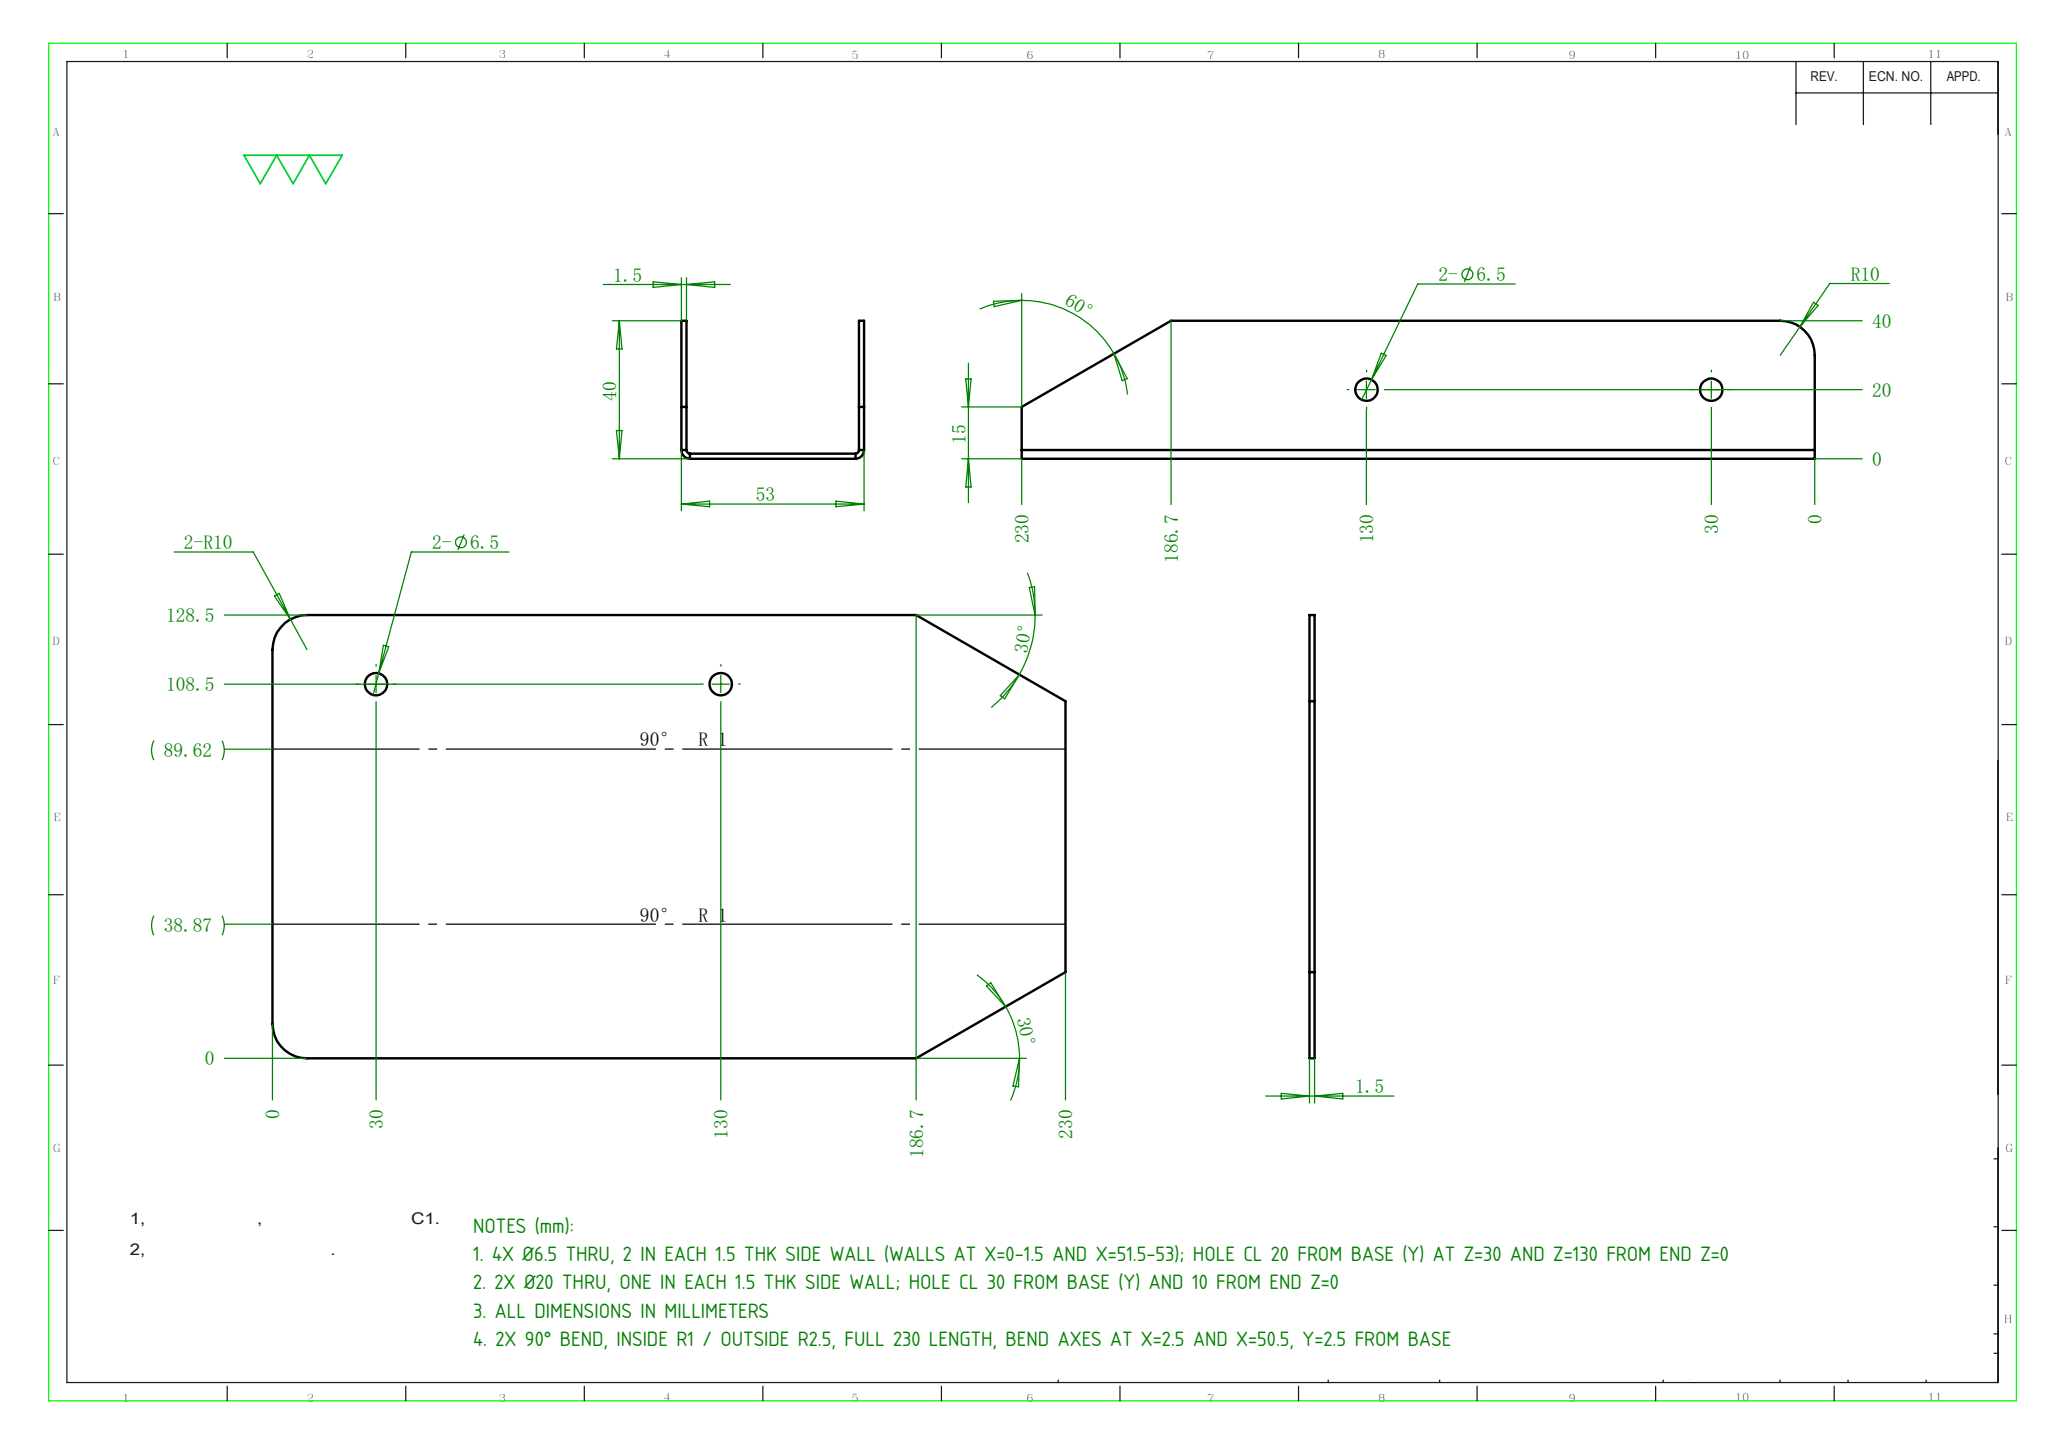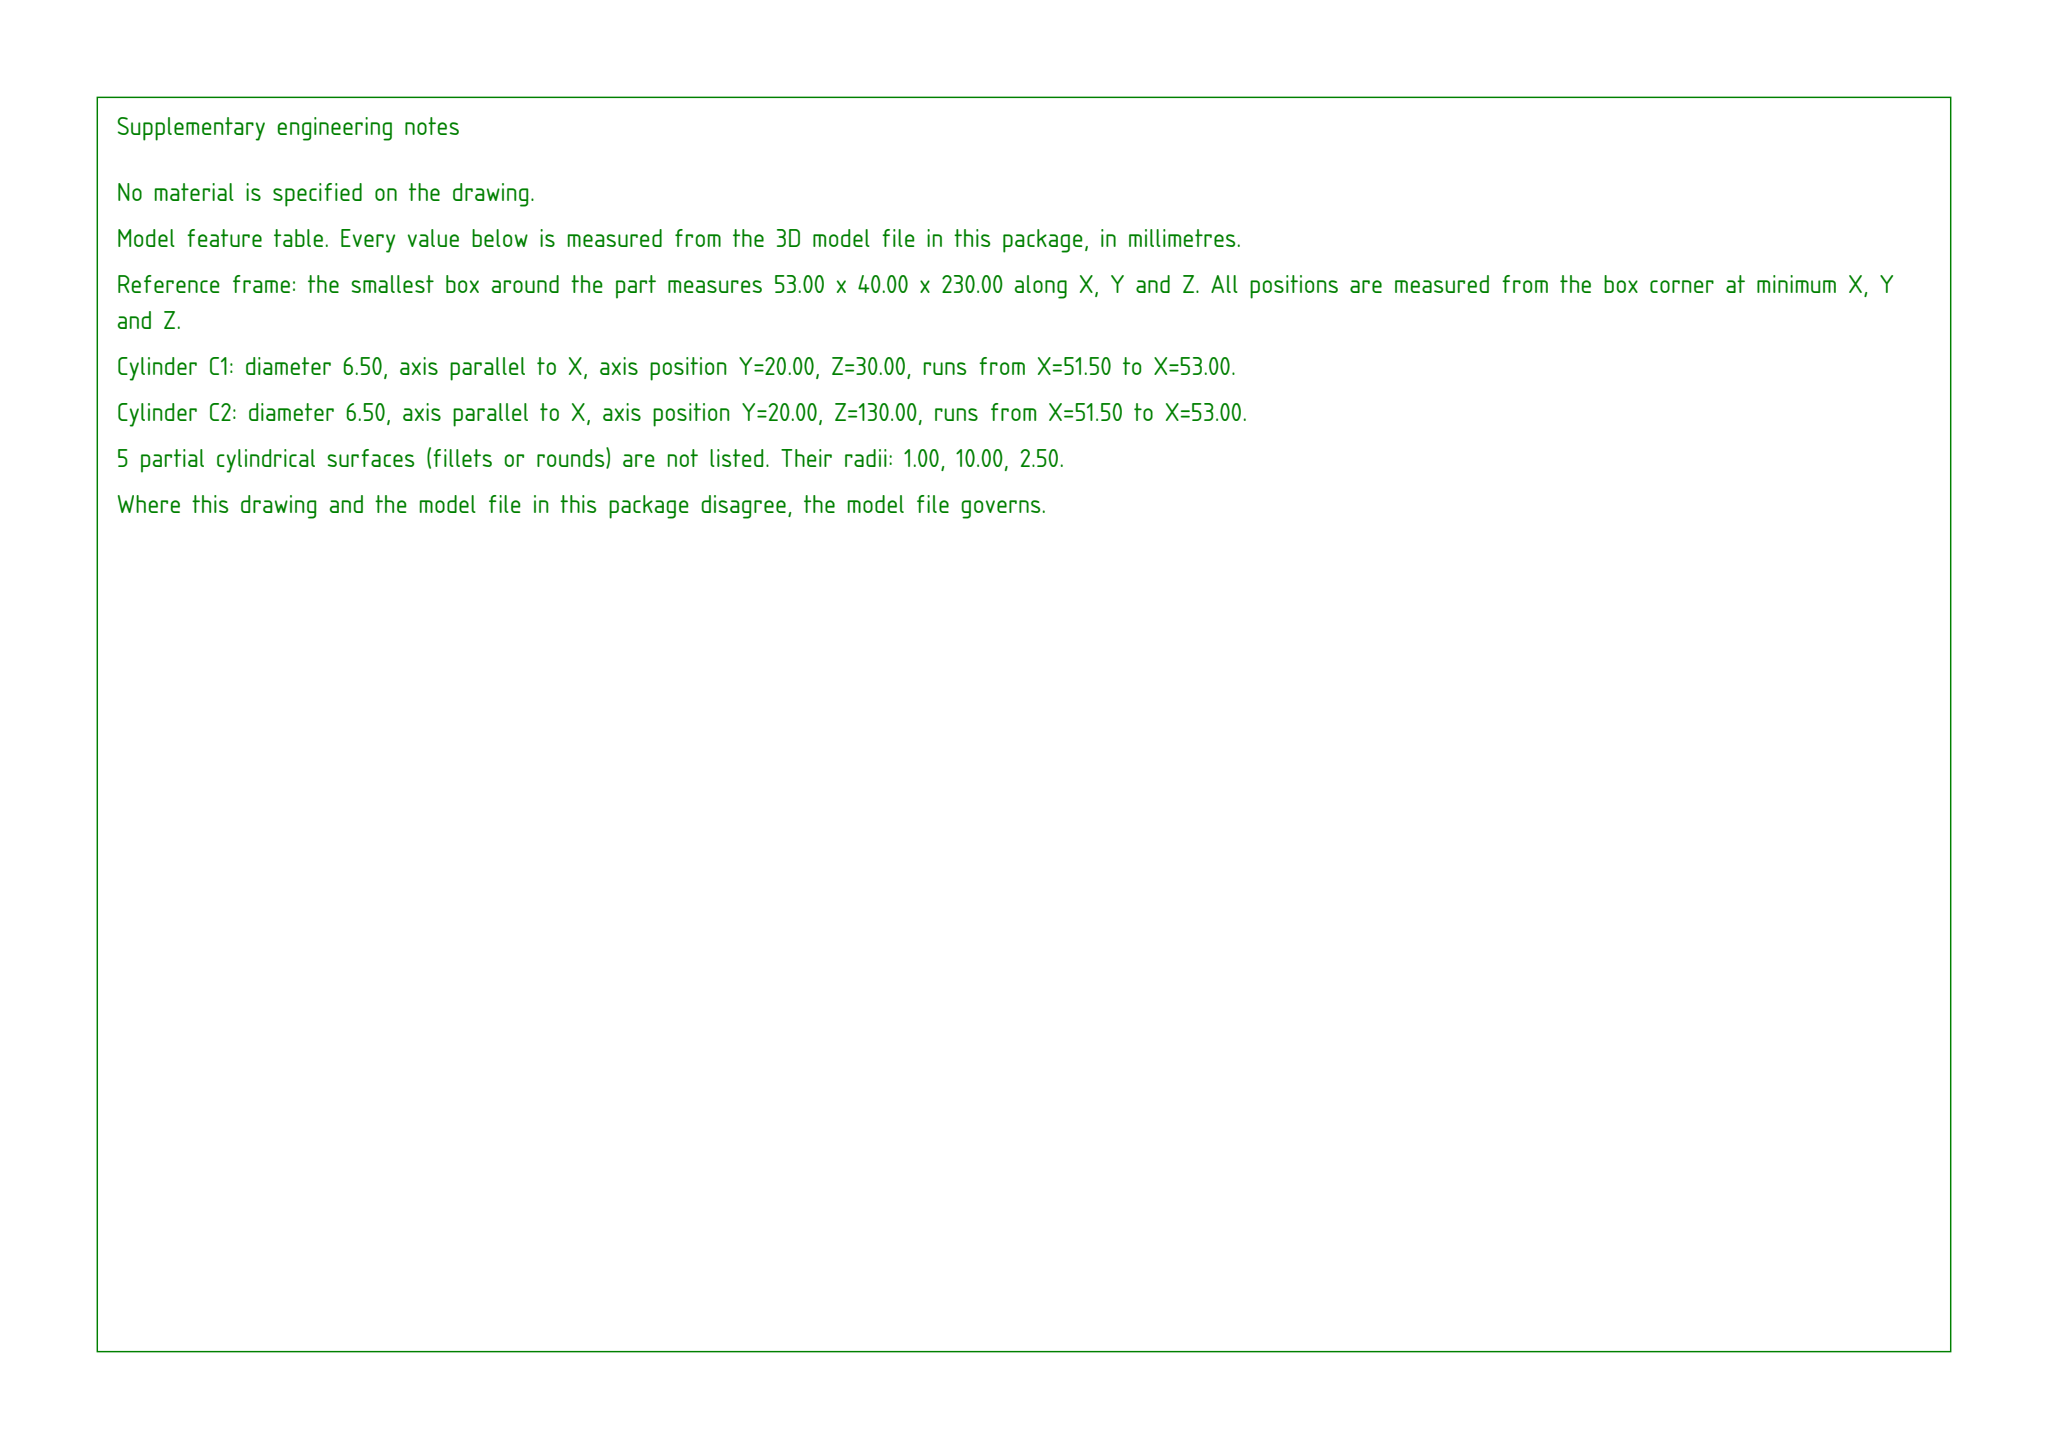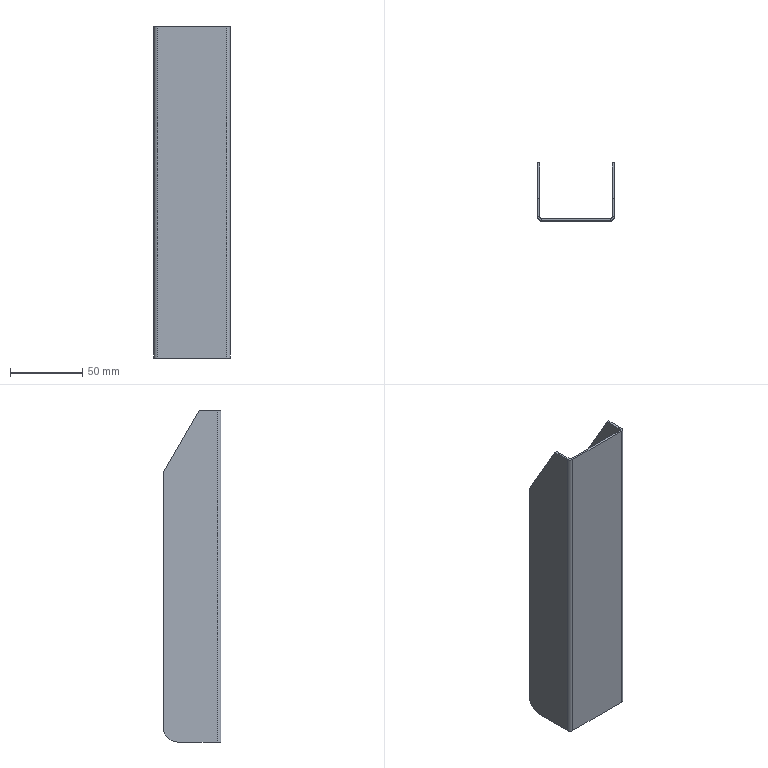Part | SolidWorks | mm | 1 solid | 30 faces | box 53 x 40 x 230 mm | volume 42544 mm3 | plane 20 | cylinder 10 | commonest cylinder face diameters 6.5 x4 2 x2 5 x2 20 x2
Drawing notes:
4X Ø6.5 THRU, 2 IN EACH 1.5 THK SIDE WALL (WALLS AT X=0-1.5 AND X=51.5-53); HOLE CL 20 FROM BASE (Y) AT Z=30 AND Z=130 FROM END Z=0 | from the solid: cylinders dia 6.5, axis x, [null,20,30] and [null,20,130], length 1.5, count 2 each
2X Ø20 THRU, ONE IN EACH 1.5 THK SIDE WALL; HOLE CL 30 FROM BASE (Y) AND 10 FROM END Z=0 | from the solid: cylinders dia 20, axis x, [null,30,10], length 1.5, count 2
ALL DIMENSIONS IN MILLIMETERS | from the solid: STEP model bbox and all feature sizes given in mm (53 x 40 x 230)
2X 90° BEND, INSIDE R1 / OUTSIDE R2.5, FULL 230 LENGTH, BEND AXES AT X=2.5 AND X=50.5, Y=2.5 FROM BASE | from the solid: cylinders dia 2.0 and dia 5.0, axis z, at (x=2.5,y=2.5) and (x=50.5,y=2.5), length 230
STEP:
#1=CARTESIAN_POINT('',(51.5,18.5,-193.25));
#2=VERTEX_POINT('',#1);
#3=CARTESIAN_POINT('',(51.5,18.5,-186.75));
#4=VERTEX_POINT('',#3);
#5=CARTESIAN_POINT('',(51.5,18.5,-190.));
#6=DIRECTION('',(-1.,0.,0.));
#7=DIRECTION('',(0.,0.,1.));
#8=AXIS2_PLACEMENT_3D('',#5,#6,#7);
#9=CIRCLE('',#8,3.25);
#10=EDGE_CURVE('',#2,#4,#9,.T.);
#11=ORIENTED_EDGE('',*,*,#10,.F.);
#12=CARTESIAN_POINT('',(50.,18.5,-193.25));
#13=VERTEX_POINT('',#12);
#14=CARTESIAN_POINT('',(50.,18.5,-193.25));
#15=DIRECTION('',(-1.,0.,0.));
#16=VECTOR('',#15,1000.);
#17=LINE('',#14,#16);
#18=EDGE_CURVE('',#2,#13,#17,.T.);
#19=ORIENTED_EDGE('',*,*,#18,.T.);
#20=CARTESIAN_POINT('',(50.,18.5,-186.75));
#21=VERTEX_POINT('',#20);
#22=CARTESIAN_POINT('',(50.,18.5,-190.));
#23=DIRECTION('',(-1.,0.,0.));
#24=DIRECTION('',(0.,0.,1.));
#25=AXIS2_PLACEMENT_3D('',#22,#23,#24);
#26=CIRCLE('',#25,3.25);
#27=EDGE_CURVE('',#13,#21,#26,.T.);
#28=ORIENTED_EDGE('',*,*,#27,.T.);
#29=CARTESIAN_POINT('',(50.,18.5,-186.75));
#30=DIRECTION('',(-1.,0.,0.));
#31=VECTOR('',#30,1000.);
#32=LINE('',#29,#31);
#33=EDGE_CURVE('',#4,#21,#32,.T.);
#34=ORIENTED_EDGE('',*,*,#33,.F.);
#35=EDGE_LOOP('',(#11,#19,#28,#34));
#36=FACE_OUTER_BOUND('',#35,.T.);
#37=CARTESIAN_POINT('',(50.,18.5,-190.));
#38=DIRECTION('',(-1.,0.,0.));
#39=DIRECTION('',(0.,0.,1.));
#40=AXIS2_PLACEMENT_3D('',#37,#38,#39);
#41=CYLINDRICAL_SURFACE('',#40,3.25);
#42=ADVANCED_FACE('',(#36),#41,.F.);
#43=CARTESIAN_POINT('',(51.5,18.5,-93.25));
#44=VERTEX_POINT('',#43);
#45=CARTESIAN_POINT('',(51.5,18.5,-86.75));
#46=VERTEX_POINT('',#45);
#47=CARTESIAN_POINT('',(51.5,18.5,-90.));
#48=DIRECTION('',(-1.,0.,0.));
#49=DIRECTION('',(0.,0.,1.));
#50=AXIS2_PLACEMENT_3D('',#47,#48,#49);
#51=CIRCLE('',#50,3.25);
#52=EDGE_CURVE('',#44,#46,#51,.T.);
#53=ORIENTED_EDGE('',*,*,#52,.F.);
#54=CARTESIAN_POINT('',(50.,18.5,-93.25));
#55=VERTEX_POINT('',#54);
#56=CARTESIAN_POINT('',(50.,18.5,-93.25));
#57=DIRECTION('',(-1.,0.,0.));
#58=VECTOR('',#57,1000.);
#59=LINE('',#56,#58);
#60=EDGE_CURVE('',#44,#55,#59,.T.);
#61=ORIENTED_EDGE('',*,*,#60,.T.);
#62=CARTESIAN_POINT('',(50.,18.5,-86.75));
#63=VERTEX_POINT('',#62);
#64=CARTESIAN_POINT('',(50.,18.5,-90.));
#65=DIRECTION('',(-1.,0.,0.));
#66=DIRECTION('',(0.,0.,1.));
#67=AXIS2_PLACEMENT_3D('',#64,#65,#66);
#68=CIRCLE('',#67,3.25);
#69=EDGE_CURVE('',#55,#63,#68,.T.);
#70=ORIENTED_EDGE('',*,*,#69,.T.);
#71=CARTESIAN_POINT('',(50.,18.5,-86.75));
#72=DIRECTION('',(-1.,0.,0.));
#73=VECTOR('',#72,1000.);
#74=LINE('',#71,#73);
#75=EDGE_CURVE('',#46,#63,#74,.T.);
#76=ORIENTED_EDGE('',*,*,#75,.F.);
#77=EDGE_LOOP('',(#53,#61,#70,#76));
#78=FACE_OUTER_BOUND('',#77,.T.);
#79=CARTESIAN_POINT('',(50.,18.5,-90.));
#80=DIRECTION('',(-1.,0.,0.));
#81=DIRECTION('',(0.,0.,1.));
#82=AXIS2_PLACEMENT_3D('',#79,#80,#81);
#83=CYLINDRICAL_SURFACE('',#82,3.25);
#84=ADVANCED_FACE('',(#78),#83,.F.);
#85=CARTESIAN_POINT('',(51.5,1.,10.));
#86=VERTEX_POINT('',#85);
#87=CARTESIAN_POINT('',(51.5,13.5,10.));
#88=VERTEX_POINT('',#87);
#89=CARTESIAN_POINT('',(51.5,0.,10.));
#90=DIRECTION('',(0.,1.,0.));
#91=VECTOR('',#90,1000.);
#92=LINE('',#89,#91);
#93=EDGE_CURVE('',#86,#88,#92,.T.);
#94=ORIENTED_EDGE('',*,*,#93,.T.);
#95=CARTESIAN_POINT('',(50.,13.5,10.));
#96=VERTEX_POINT('',#95);
#97=CARTESIAN_POINT('',(50.,13.5,10.));
#98=DIRECTION('',(1.,0.,0.));
#99=VECTOR('',#98,1000.);
#100=LINE('',#97,#99);
#101=EDGE_CURVE('',#96,#88,#100,.T.);
#102=ORIENTED_EDGE('',*,*,#101,.F.);
#103=CARTESIAN_POINT('',(50.,1.,10.));
#104=VERTEX_POINT('',#103);
#105=CARTESIAN_POINT('',(50.,0.,10.));
#106=DIRECTION('',(0.,1.,0.));
#107=VECTOR('',#106,1000.);
#108=LINE('',#105,#107);
#109=EDGE_CURVE('',#104,#96,#108,.T.);
#110=ORIENTED_EDGE('',*,*,#109,.F.);
#111=CARTESIAN_POINT('',(50.,1.,10.));
#112=DIRECTION('',(1.,0.,0.));
#113=VECTOR('',#112,1000.);
#114=LINE('',#111,#113);
#115=EDGE_CURVE('',#104,#86,#114,.T.);
#116=ORIENTED_EDGE('',*,*,#115,.T.);
#117=EDGE_LOOP('',(#94,#102,#110,#116));
#118=FACE_OUTER_BOUND('',#117,.T.);
#119=CARTESIAN_POINT('',(49.,-1.5,10.));
#120=DIRECTION('',(0.,0.,1.));
#121=DIRECTION('',(1.,0.,0.));
#122=AXIS2_PLACEMENT_3D('',#119,#120,#121);
#123=PLANE('',#122);
#124=ADVANCED_FACE('',(#118),#123,.T.);
#125=CARTESIAN_POINT('',(51.5,18.5,-90.));
#126=DIRECTION('',(-1.,0.,0.));
#127=DIRECTION('',(0.,0.,1.));
#128=AXIS2_PLACEMENT_3D('',#125,#126,#127);
#129=CIRCLE('',#128,3.25);
#130=EDGE_CURVE('',#46,#44,#129,.T.);
#131=ORIENTED_EDGE('',*,*,#130,.T.);
#132=ORIENTED_EDGE('',*,*,#52,.T.);
#133=EDGE_LOOP('',(#131,#132));
#134=FACE_BOUND('',#133,.T.);
#135=CARTESIAN_POINT('',(51.5,18.5,-190.));
#136=DIRECTION('',(-1.,0.,0.));
#137=DIRECTION('',(0.,0.,1.));
#138=AXIS2_PLACEMENT_3D('',#135,#136,#137);
#139=CIRCLE('',#138,3.25);
#140=EDGE_CURVE('',#4,#2,#139,.T.);
#141=ORIENTED_EDGE('',*,*,#140,.T.);
#142=ORIENTED_EDGE('',*,*,#10,.T.);
#143=EDGE_LOOP('',(#141,#142));
#144=FACE_BOUND('',#143,.T.);
#145=CARTESIAN_POINT('',(51.5,38.5,-33.301));
#146=VERTEX_POINT('',#145);
#147=CARTESIAN_POINT('',(51.5,10.125,15.846));
#148=DIRECTION('',(0.,-0.5,0.866));
#149=VECTOR('',#148,1000.);
#150=LINE('',#147,#149);
#151=EDGE_CURVE('',#146,#88,#150,.T.);
#152=ORIENTED_EDGE('',*,*,#151,.T.);
#153=ORIENTED_EDGE('',*,*,#93,.F.);
#154=CARTESIAN_POINT('',(51.5,1.,-220.));
#155=VERTEX_POINT('',#154);
#156=CARTESIAN_POINT('',(51.5,1.,10.));
#157=DIRECTION('',(0.,0.,-1.));
#158=VECTOR('',#157,1000.);
#159=LINE('',#156,#158);
#160=EDGE_CURVE('',#86,#155,#159,.T.);
#161=ORIENTED_EDGE('',*,*,#160,.T.);
#162=CARTESIAN_POINT('',(51.5,28.5,-220.));
#163=VERTEX_POINT('',#162);
#164=CARTESIAN_POINT('',(51.5,0.,-220.));
#165=DIRECTION('',(0.,1.,0.));
#166=VECTOR('',#165,1000.);
#167=LINE('',#164,#166);
#168=EDGE_CURVE('',#155,#163,#167,.T.);
#169=ORIENTED_EDGE('',*,*,#168,.T.);
#170=CARTESIAN_POINT('',(51.5,38.5,-210.));
#171=VERTEX_POINT('',#170);
#172=CARTESIAN_POINT('',(51.5,28.5,-210.));
#173=DIRECTION('',(1.,0.,0.));
#174=DIRECTION('',(0.,0.,1.));
#175=AXIS2_PLACEMENT_3D('',#172,#173,#174);
#176=CIRCLE('',#175,10.);
#177=EDGE_CURVE('',#163,#171,#176,.T.);
#178=ORIENTED_EDGE('',*,*,#177,.T.);
#179=CARTESIAN_POINT('',(51.5,38.5,10.));
#180=DIRECTION('',(0.,0.,-1.));
#181=VECTOR('',#180,1000.);
#182=LINE('',#179,#181);
#183=EDGE_CURVE('',#146,#171,#182,.T.);
#184=ORIENTED_EDGE('',*,*,#183,.F.);
#185=EDGE_LOOP('',(#152,#153,#161,#169,#178,#184));
#186=FACE_OUTER_BOUND('',#185,.T.);
#187=CARTESIAN_POINT('',(51.5,0.,10.));
#188=DIRECTION('',(-1.,0.,0.));
#189=DIRECTION('',(0.,0.,1.));
#190=AXIS2_PLACEMENT_3D('',#187,#188,#189);
#191=PLANE('',#190);
#192=ADVANCED_FACE('',(#134,#144,#186),#191,.F.);
#193=CARTESIAN_POINT('',(50.,38.5,-33.301));
#194=VERTEX_POINT('',#193);
#195=CARTESIAN_POINT('',(50.,38.5,-210.));
#196=VERTEX_POINT('',#195);
#197=CARTESIAN_POINT('',(50.,38.5,10.));
#198=DIRECTION('',(0.,0.,-1.));
#199=VECTOR('',#198,1000.);
#200=LINE('',#197,#199);
#201=EDGE_CURVE('',#194,#196,#200,.T.);
#202=ORIENTED_EDGE('',*,*,#201,.F.);
#203=CARTESIAN_POINT('',(50.,38.5,-33.301));
#204=DIRECTION('',(1.,0.,0.));
#205=VECTOR('',#204,1000.);
#206=LINE('',#203,#205);
#207=EDGE_CURVE('',#194,#146,#206,.T.);
#208=ORIENTED_EDGE('',*,*,#207,.T.);
#209=ORIENTED_EDGE('',*,*,#183,.T.);
#210=CARTESIAN_POINT('',(50.,38.5,-210.));
#211=DIRECTION('',(-1.,0.,0.));
#212=VECTOR('',#211,1000.);
#213=LINE('',#210,#212);
#214=EDGE_CURVE('',#171,#196,#213,.T.);
#215=ORIENTED_EDGE('',*,*,#214,.T.);
#216=EDGE_LOOP('',(#202,#208,#209,#215));
#217=FACE_OUTER_BOUND('',#216,.T.);
#218=CARTESIAN_POINT('',(50.,38.5,10.));
#219=DIRECTION('',(0.,1.,0.));
#220=DIRECTION('',(0.,0.,1.));
#221=AXIS2_PLACEMENT_3D('',#218,#219,#220);
#222=PLANE('',#221);
#223=ADVANCED_FACE('',(#217),#222,.T.);
#224=CARTESIAN_POINT('',(50.,18.5,-90.));
#225=DIRECTION('',(-1.,0.,0.));
#226=DIRECTION('',(0.,0.,1.));
#227=AXIS2_PLACEMENT_3D('',#224,#225,#226);
#228=CIRCLE('',#227,3.25);
#229=EDGE_CURVE('',#63,#55,#228,.T.);
#230=ORIENTED_EDGE('',*,*,#229,.F.);
#231=ORIENTED_EDGE('',*,*,#69,.F.);
#232=EDGE_LOOP('',(#230,#231));
#233=FACE_BOUND('',#232,.T.);
#234=CARTESIAN_POINT('',(50.,18.5,-190.));
#235=DIRECTION('',(-1.,0.,0.));
#236=DIRECTION('',(0.,0.,1.));
#237=AXIS2_PLACEMENT_3D('',#234,#235,#236);
#238=CIRCLE('',#237,3.25);
#239=EDGE_CURVE('',#21,#13,#238,.T.);
#240=ORIENTED_EDGE('',*,*,#239,.F.);
#241=ORIENTED_EDGE('',*,*,#27,.F.);
#242=EDGE_LOOP('',(#240,#241));
#243=FACE_BOUND('',#242,.T.);
#244=ORIENTED_EDGE('',*,*,#109,.T.);
#245=CARTESIAN_POINT('',(50.,10.125,15.846));
#246=DIRECTION('',(0.,-0.5,0.866));
#247=VECTOR('',#246,1000.);
#248=LINE('',#245,#247);
#249=EDGE_CURVE('',#194,#96,#248,.T.);
#250=ORIENTED_EDGE('',*,*,#249,.F.);
#251=ORIENTED_EDGE('',*,*,#201,.T.);
#252=CARTESIAN_POINT('',(50.,28.5,-220.));
#253=VERTEX_POINT('',#252);
#254=CARTESIAN_POINT('',(50.,28.5,-210.));
#255=DIRECTION('',(-1.,0.,0.));
#256=DIRECTION('',(0.,0.,1.));
#257=AXIS2_PLACEMENT_3D('',#254,#255,#256);
#258=CIRCLE('',#257,10.);
#259=EDGE_CURVE('',#196,#253,#258,.T.);
#260=ORIENTED_EDGE('',*,*,#259,.T.);
#261=CARTESIAN_POINT('',(50.,1.,-220.));
#262=VERTEX_POINT('',#261);
#263=CARTESIAN_POINT('',(50.,0.,-220.));
#264=DIRECTION('',(0.,1.,0.));
#265=VECTOR('',#264,1000.);
#266=LINE('',#263,#265);
#267=EDGE_CURVE('',#262,#253,#266,.T.);
#268=ORIENTED_EDGE('',*,*,#267,.F.);
#269=CARTESIAN_POINT('',(50.,1.,10.));
#270=DIRECTION('',(0.,0.,-1.));
#271=VECTOR('',#270,1000.);
#272=LINE('',#269,#271);
#273=EDGE_CURVE('',#104,#262,#272,.T.);
#274=ORIENTED_EDGE('',*,*,#273,.F.);
#275=EDGE_LOOP('',(#244,#250,#251,#260,#268,#274));
#276=FACE_OUTER_BOUND('',#275,.T.);
#277=CARTESIAN_POINT('',(50.,0.,10.));
#278=DIRECTION('',(-1.,0.,0.));
#279=DIRECTION('',(0.,0.,1.));
#280=AXIS2_PLACEMENT_3D('',#277,#278,#279);
#281=PLANE('',#280);
#282=ADVANCED_FACE('',(#233,#243,#276),#281,.T.);
#283=CARTESIAN_POINT('',(0.,38.5,-33.301));
#284=VERTEX_POINT('',#283);
#285=CARTESIAN_POINT('',(0.,38.5,-210.));
#286=VERTEX_POINT('',#285);
#287=CARTESIAN_POINT('',(0.,38.5,10.));
#288=DIRECTION('',(0.,0.,-1.));
#289=VECTOR('',#288,1000.);
#290=LINE('',#287,#289);
#291=EDGE_CURVE('',#284,#286,#290,.T.);
#292=ORIENTED_EDGE('',*,*,#291,.F.);
#293=CARTESIAN_POINT('',(0.,13.5,10.));
#294=VERTEX_POINT('',#293);
#295=CARTESIAN_POINT('',(0.,10.125,15.846));
#296=DIRECTION('',(0.,0.5,-0.866));
#297=VECTOR('',#296,1000.);
#298=LINE('',#295,#297);
#299=EDGE_CURVE('',#294,#284,#298,.T.);
#300=ORIENTED_EDGE('',*,*,#299,.F.);
#301=CARTESIAN_POINT('',(0.,1.,10.));
#302=VERTEX_POINT('',#301);
#303=CARTESIAN_POINT('',(0.,0.,10.));
#304=DIRECTION('',(0.,-1.,0.));
#305=VECTOR('',#304,1000.);
#306=LINE('',#303,#305);
#307=EDGE_CURVE('',#294,#302,#306,.T.);
#308=ORIENTED_EDGE('',*,*,#307,.T.);
#309=CARTESIAN_POINT('',(0.,1.,-220.));
#310=VERTEX_POINT('',#309);
#311=CARTESIAN_POINT('',(0.,1.,10.));
#312=DIRECTION('',(0.,0.,-1.));
#313=VECTOR('',#312,1000.);
#314=LINE('',#311,#313);
#315=EDGE_CURVE('',#302,#310,#314,.T.);
#316=ORIENTED_EDGE('',*,*,#315,.T.);
#317=CARTESIAN_POINT('',(0.,28.5,-220.));
#318=VERTEX_POINT('',#317);
#319=CARTESIAN_POINT('',(0.,0.,-220.));
#320=DIRECTION('',(0.,-1.,0.));
#321=VECTOR('',#320,1000.);
#322=LINE('',#319,#321);
#323=EDGE_CURVE('',#318,#310,#322,.T.);
#324=ORIENTED_EDGE('',*,*,#323,.F.);
#325=CARTESIAN_POINT('',(0.,28.5,-210.));
#326=DIRECTION('',(1.,0.,0.));
#327=DIRECTION('',(0.,0.,-1.));
#328=AXIS2_PLACEMENT_3D('',#325,#326,#327);
#329=CIRCLE('',#328,10.);
#330=EDGE_CURVE('',#318,#286,#329,.T.);
#331=ORIENTED_EDGE('',*,*,#330,.T.);
#332=EDGE_LOOP('',(#292,#300,#308,#316,#324,#331));
#333=FACE_OUTER_BOUND('',#332,.T.);
#334=CARTESIAN_POINT('',(0.,0.,10.));
#335=DIRECTION('',(1.,0.,0.));
#336=DIRECTION('',(0.,0.,-1.));
#337=AXIS2_PLACEMENT_3D('',#334,#335,#336);
#338=PLANE('',#337);
#339=ADVANCED_FACE('',(#333),#338,.T.);
#340=CARTESIAN_POINT('',(-1.5,38.5,-33.301));
#341=VERTEX_POINT('',#340);
#342=CARTESIAN_POINT('',(-1.5,38.5,-210.));
#343=VERTEX_POINT('',#342);
#344=CARTESIAN_POINT('',(-1.5,38.5,10.));
#345=DIRECTION('',(0.,0.,-1.));
#346=VECTOR('',#345,1000.);
#347=LINE('',#344,#346);
#348=EDGE_CURVE('',#341,#343,#347,.T.);
#349=ORIENTED_EDGE('',*,*,#348,.F.);
#350=CARTESIAN_POINT('',(0.,38.5,-33.301));
#351=DIRECTION('',(-1.,0.,0.));
#352=VECTOR('',#351,1000.);
#353=LINE('',#350,#352);
#354=EDGE_CURVE('',#284,#341,#353,.T.);
#355=ORIENTED_EDGE('',*,*,#354,.F.);
#356=ORIENTED_EDGE('',*,*,#291,.T.);
#357=CARTESIAN_POINT('',(-1.5,38.5,-210.));
#358=DIRECTION('',(-1.,0.,0.));
#359=VECTOR('',#358,1000.);
#360=LINE('',#357,#359);
#361=EDGE_CURVE('',#286,#343,#360,.T.);
#362=ORIENTED_EDGE('',*,*,#361,.T.);
#363=EDGE_LOOP('',(#349,#355,#356,#362));
#364=FACE_OUTER_BOUND('',#363,.T.);
#365=CARTESIAN_POINT('',(-1.5,38.5,10.));
#366=DIRECTION('',(0.,1.,0.));
#367=DIRECTION('',(0.,0.,1.));
#368=AXIS2_PLACEMENT_3D('',#365,#366,#367);
#369=PLANE('',#368);
#370=ADVANCED_FACE('',(#364),#369,.T.);
#371=CARTESIAN_POINT('',(-1.5,13.5,10.));
#372=VERTEX_POINT('',#371);
#373=CARTESIAN_POINT('',(-1.5,10.125,15.846));
#374=DIRECTION('',(0.,0.5,-0.866));
#375=VECTOR('',#374,1000.);
#376=LINE('',#373,#375);
#377=EDGE_CURVE('',#372,#341,#376,.T.);
#378=ORIENTED_EDGE('',*,*,#377,.T.);
#379=ORIENTED_EDGE('',*,*,#348,.T.);
#380=CARTESIAN_POINT('',(-1.5,28.5,-220.));
#381=VERTEX_POINT('',#380);
#382=CARTESIAN_POINT('',(-1.5,28.5,-210.));
#383=DIRECTION('',(-1.,0.,0.));
#384=DIRECTION('',(0.,0.,-1.));
#385=AXIS2_PLACEMENT_3D('',#382,#383,#384);
#386=CIRCLE('',#385,10.);
#387=EDGE_CURVE('',#343,#381,#386,.T.);
#388=ORIENTED_EDGE('',*,*,#387,.T.);
#389=CARTESIAN_POINT('',(-1.5,1.,-220.));
#390=VERTEX_POINT('',#389);
#391=CARTESIAN_POINT('',(-1.5,0.,-220.));
#392=DIRECTION('',(0.,-1.,0.));
#393=VECTOR('',#392,1000.);
#394=LINE('',#391,#393);
#395=EDGE_CURVE('',#381,#390,#394,.T.);
#396=ORIENTED_EDGE('',*,*,#395,.T.);
#397=CARTESIAN_POINT('',(-1.5,1.,10.));
#398=VERTEX_POINT('',#397);
#399=CARTESIAN_POINT('',(-1.5,1.,10.));
#400=DIRECTION('',(0.,0.,-1.));
#401=VECTOR('',#400,1000.);
#402=LINE('',#399,#401);
#403=EDGE_CURVE('',#398,#390,#402,.T.);
#404=ORIENTED_EDGE('',*,*,#403,.F.);
#405=CARTESIAN_POINT('',(-1.5,0.,10.));
#406=DIRECTION('',(0.,-1.,0.));
#407=VECTOR('',#406,1000.);
#408=LINE('',#405,#407);
#409=EDGE_CURVE('',#372,#398,#408,.T.);
#410=ORIENTED_EDGE('',*,*,#409,.F.);
#411=EDGE_LOOP('',(#378,#379,#388,#396,#404,#410));
#412=FACE_OUTER_BOUND('',#411,.T.);
#413=CARTESIAN_POINT('',(-1.5,0.,10.));
#414=DIRECTION('',(1.,0.,0.));
#415=DIRECTION('',(0.,0.,-1.));
#416=AXIS2_PLACEMENT_3D('',#413,#414,#415);
#417=PLANE('',#416);
#418=ADVANCED_FACE('',(#412),#417,.F.);
#419=CARTESIAN_POINT('',(0.,13.5,10.));
#420=DIRECTION('',(-1.,0.,0.));
#421=VECTOR('',#420,1000.);
#422=LINE('',#419,#421);
#423=EDGE_CURVE('',#294,#372,#422,.T.);
#424=ORIENTED_EDGE('',*,*,#423,.T.);
#425=ORIENTED_EDGE('',*,*,#409,.T.);
#426=CARTESIAN_POINT('',(-1.5,1.,10.));
#427=DIRECTION('',(1.,-0.,0.));
#428=VECTOR('',#427,1000.);
#429=LINE('',#426,#428);
#430=EDGE_CURVE('',#398,#302,#429,.T.);
#431=ORIENTED_EDGE('',*,*,#430,.T.);
#432=ORIENTED_EDGE('',*,*,#307,.F.);
#433=EDGE_LOOP('',(#424,#425,#431,#432));
#434=FACE_OUTER_BOUND('',#433,.T.);
#435=CARTESIAN_POINT('',(49.,1.,10.));
#436=DIRECTION('',(0.,0.,-1.));
#437=DIRECTION('',(-1.,0.,0.));
#438=AXIS2_PLACEMENT_3D('',#435,#436,#437);
#439=PLANE('',#438);
#440=ADVANCED_FACE('',(#434),#439,.F.);
#441=CARTESIAN_POINT('',(1.,0.,10.));
#442=VERTEX_POINT('',#441);
#443=CARTESIAN_POINT('',(1.,-1.5,10.));
#444=VERTEX_POINT('',#443);
#445=CARTESIAN_POINT('',(1.,0.,10.));
#446=DIRECTION('',(0.,-1.,0.));
#447=VECTOR('',#446,1000.);
#448=LINE('',#445,#447);
#449=EDGE_CURVE('',#442,#444,#448,.T.);
#450=ORIENTED_EDGE('',*,*,#449,.F.);
#451=CARTESIAN_POINT('',(1.,1.,10.));
#452=DIRECTION('',(0.,0.,1.));
#453=DIRECTION('',(-1.,0.,0.));
#454=AXIS2_PLACEMENT_3D('',#451,#452,#453);
#455=CIRCLE('',#454,1.);
#456=EDGE_CURVE('',#302,#442,#455,.T.);
#457=ORIENTED_EDGE('',*,*,#456,.F.);
#458=ORIENTED_EDGE('',*,*,#430,.F.);
#459=CARTESIAN_POINT('',(1.,1.,10.));
#460=DIRECTION('',(0.,0.,1.));
#461=DIRECTION('',(1.,0.,0.));
#462=AXIS2_PLACEMENT_3D('',#459,#460,#461);
#463=CIRCLE('',#462,2.5);
#464=EDGE_CURVE('',#398,#444,#463,.T.);
#465=ORIENTED_EDGE('',*,*,#464,.T.);
#466=EDGE_LOOP('',(#450,#457,#458,#465));
#467=FACE_OUTER_BOUND('',#466,.T.);
#468=CARTESIAN_POINT('',(1.,0.,10.));
#469=DIRECTION('',(0.,0.,1.));
#470=DIRECTION('',(1.,0.,0.));
#471=AXIS2_PLACEMENT_3D('',#468,#469,#470);
#472=PLANE('',#471);
#473=ADVANCED_FACE('',(#467),#472,.T.);
#474=CARTESIAN_POINT('',(49.,0.,10.));
#475=VERTEX_POINT('',#474);
#476=CARTESIAN_POINT('',(0.,0.,10.));
#477=DIRECTION('',(1.,0.,0.));
#478=VECTOR('',#477,1000.);
#479=LINE('',#476,#478);
#480=EDGE_CURVE('',#442,#475,#479,.T.);
#481=ORIENTED_EDGE('',*,*,#480,.F.);
#482=ORIENTED_EDGE('',*,*,#449,.T.);
#483=CARTESIAN_POINT('',(49.,-1.5,10.));
#484=VERTEX_POINT('',#483);
#485=CARTESIAN_POINT('',(0.,-1.5,10.));
#486=DIRECTION('',(1.,0.,0.));
#487=VECTOR('',#486,1000.);
#488=LINE('',#485,#487);
#489=EDGE_CURVE('',#444,#484,#488,.T.);
#490=ORIENTED_EDGE('',*,*,#489,.T.);
#491=CARTESIAN_POINT('',(49.,-1.5,10.));
#492=DIRECTION('',(0.,1.,0.));
#493=VECTOR('',#492,1000.);
#494=LINE('',#491,#493);
#495=EDGE_CURVE('',#484,#475,#494,.T.);
#496=ORIENTED_EDGE('',*,*,#495,.T.);
#497=EDGE_LOOP('',(#481,#482,#490,#496));
#498=FACE_OUTER_BOUND('',#497,.T.);
#499=CARTESIAN_POINT('',(-1.5,1.,10.));
#500=DIRECTION('',(0.,0.,1.));
#501=DIRECTION('',(1.,0.,0.));
#502=AXIS2_PLACEMENT_3D('',#499,#500,#501);
#503=PLANE('',#502);
#504=ADVANCED_FACE('',(#498),#503,.T.);
#505=CARTESIAN_POINT('',(0.,1.,-220.));
#506=DIRECTION('',(-1.,0.,0.));
#507=VECTOR('',#506,1000.);
#508=LINE('',#505,#507);
#509=EDGE_CURVE('',#310,#390,#508,.T.);
#510=ORIENTED_EDGE('',*,*,#509,.F.);
#511=CARTESIAN_POINT('',(1.,0.,-220.));
#512=VERTEX_POINT('',#511);
#513=CARTESIAN_POINT('',(1.,1.,-220.));
#514=DIRECTION('',(0.,0.,1.));
#515=DIRECTION('',(-1.,0.,0.));
#516=AXIS2_PLACEMENT_3D('',#513,#514,#515);
#517=CIRCLE('',#516,1.);
#518=EDGE_CURVE('',#310,#512,#517,.T.);
#519=ORIENTED_EDGE('',*,*,#518,.T.);
#520=CARTESIAN_POINT('',(1.,-1.5,-220.));
#521=VERTEX_POINT('',#520);
#522=CARTESIAN_POINT('',(1.,-1.5,-220.));
#523=DIRECTION('',(0.,1.,0.));
#524=VECTOR('',#523,1000.);
#525=LINE('',#522,#524);
#526=EDGE_CURVE('',#521,#512,#525,.T.);
#527=ORIENTED_EDGE('',*,*,#526,.F.);
#528=CARTESIAN_POINT('',(1.,1.,-220.));
#529=DIRECTION('',(0.,0.,1.));
#530=DIRECTION('',(1.,0.,0.));
#531=AXIS2_PLACEMENT_3D('',#528,#529,#530);
#532=CIRCLE('',#531,2.5);
#533=EDGE_CURVE('',#390,#521,#532,.T.);
#534=ORIENTED_EDGE('',*,*,#533,.F.);
#535=EDGE_LOOP('',(#510,#519,#527,#534));
#536=FACE_OUTER_BOUND('',#535,.T.);
#537=CARTESIAN_POINT('',(0.,1.,-220.));
#538=DIRECTION('',(0.,0.,-1.));
#539=DIRECTION('',(-1.,0.,0.));
#540=AXIS2_PLACEMENT_3D('',#537,#538,#539);
#541=PLANE('',#540);
#542=ADVANCED_FACE('',(#536),#541,.T.);
#543=ORIENTED_EDGE('',*,*,#395,.F.);
#544=CARTESIAN_POINT('',(1.,28.5,-220.));
#545=DIRECTION('',(1.,0.,0.));
#546=VECTOR('',#545,1000.);
#547=LINE('',#544,#546);
#548=EDGE_CURVE('',#381,#318,#547,.T.);
#549=ORIENTED_EDGE('',*,*,#548,.T.);
#550=ORIENTED_EDGE('',*,*,#323,.T.);
#551=ORIENTED_EDGE('',*,*,#509,.T.);
#552=EDGE_LOOP('',(#543,#549,#550,#551));
#553=FACE_OUTER_BOUND('',#552,.T.);
#554=CARTESIAN_POINT('',(1.,-1.5,-220.));
#555=DIRECTION('',(0.,0.,-1.));
#556=DIRECTION('',(-1.,0.,0.));
#557=AXIS2_PLACEMENT_3D('',#554,#555,#556);
#558=PLANE('',#557);
#559=ADVANCED_FACE('',(#553),#558,.T.);
#560=ORIENTED_EDGE('',*,*,#115,.F.);
#561=CARTESIAN_POINT('',(49.,1.,10.));
#562=DIRECTION('',(0.,0.,1.));
#563=DIRECTION('',(-1.,0.,0.));
#564=AXIS2_PLACEMENT_3D('',#561,#562,#563);
#565=CIRCLE('',#564,1.);
#566=EDGE_CURVE('',#475,#104,#565,.T.);
#567=ORIENTED_EDGE('',*,*,#566,.F.);
#568=ORIENTED_EDGE('',*,*,#495,.F.);
#569=CARTESIAN_POINT('',(49.,1.,10.));
#570=DIRECTION('',(0.,0.,1.));
#571=DIRECTION('',(1.,0.,0.));
#572=AXIS2_PLACEMENT_3D('',#569,#570,#571);
#573=CIRCLE('',#572,2.5);
#574=EDGE_CURVE('',#484,#86,#573,.T.);
#575=ORIENTED_EDGE('',*,*,#574,.T.);
#576=EDGE_LOOP('',(#560,#567,#568,#575));
#577=FACE_OUTER_BOUND('',#576,.T.);
#578=CARTESIAN_POINT('',(50.,1.,10.));
#579=DIRECTION('',(0.,0.,1.));
#580=DIRECTION('',(1.,0.,0.));
#581=AXIS2_PLACEMENT_3D('',#578,#579,#580);
#582=PLANE('',#581);
#583=ADVANCED_FACE('',(#577),#582,.T.);
#584=CARTESIAN_POINT('',(49.,0.,-220.));
#585=VERTEX_POINT('',#584);
#586=CARTESIAN_POINT('',(49.,-1.5,-220.));
#587=VERTEX_POINT('',#586);
#588=CARTESIAN_POINT('',(49.,0.,-220.));
#589=DIRECTION('',(0.,-1.,0.));
#590=VECTOR('',#589,1000.);
#591=LINE('',#588,#590);
#592=EDGE_CURVE('',#585,#587,#591,.T.);
#593=ORIENTED_EDGE('',*,*,#592,.F.);
#594=CARTESIAN_POINT('',(49.,1.,-220.));
#595=DIRECTION('',(0.,0.,1.));
#596=DIRECTION('',(-1.,0.,0.));
#597=AXIS2_PLACEMENT_3D('',#594,#595,#596);
#598=CIRCLE('',#597,1.);
#599=EDGE_CURVE('',#585,#262,#598,.T.);
#600=ORIENTED_EDGE('',*,*,#599,.T.);
#601=CARTESIAN_POINT('',(51.5,1.,-220.));
#602=DIRECTION('',(-1.,0.,0.));
#603=VECTOR('',#602,1000.);
#604=LINE('',#601,#603);
#605=EDGE_CURVE('',#155,#262,#604,.T.);
#606=ORIENTED_EDGE('',*,*,#605,.F.);
#607=CARTESIAN_POINT('',(49.,1.,-220.));
#608=DIRECTION('',(0.,0.,1.));
#609=DIRECTION('',(1.,0.,0.));
#610=AXIS2_PLACEMENT_3D('',#607,#608,#609);
#611=CIRCLE('',#610,2.5);
#612=EDGE_CURVE('',#587,#155,#611,.T.);
#613=ORIENTED_EDGE('',*,*,#612,.F.);
#614=EDGE_LOOP('',(#593,#600,#606,#613));
#615=FACE_OUTER_BOUND('',#614,.T.);
#616=CARTESIAN_POINT('',(49.,0.,-220.));
#617=DIRECTION('',(0.,0.,-1.));
#618=DIRECTION('',(-1.,0.,0.));
#619=AXIS2_PLACEMENT_3D('',#616,#617,#618);
#620=PLANE('',#619);
#621=ADVANCED_FACE('',(#615),#620,.T.);
#622=CARTESIAN_POINT('',(0.,0.,-220.));
#623=DIRECTION('',(1.,0.,0.));
#624=VECTOR('',#623,1000.);
#625=LINE('',#622,#624);
#626=EDGE_CURVE('',#512,#585,#625,.T.);
#627=ORIENTED_EDGE('',*,*,#626,.T.);
#628=ORIENTED_EDGE('',*,*,#592,.T.);
#629=CARTESIAN_POINT('',(0.,-1.5,-220.));
#630=DIRECTION('',(1.,0.,0.));
#631=VECTOR('',#630,1000.);
#632=LINE('',#629,#631);
#633=EDGE_CURVE('',#521,#587,#632,.T.);
#634=ORIENTED_EDGE('',*,*,#633,.F.);
#635=ORIENTED_EDGE('',*,*,#526,.T.);
#636=EDGE_LOOP('',(#627,#628,#634,#635));
#637=FACE_OUTER_BOUND('',#636,.T.);
#638=CARTESIAN_POINT('',(51.5,1.,-220.));
#639=DIRECTION('',(0.,0.,-1.));
#640=DIRECTION('',(-1.,0.,0.));
#641=AXIS2_PLACEMENT_3D('',#638,#639,#640);
#642=PLANE('',#641);
#643=ADVANCED_FACE('',(#637),#642,.T.);
#644=ORIENTED_EDGE('',*,*,#273,.T.);
#645=ORIENTED_EDGE('',*,*,#599,.F.);
#646=CARTESIAN_POINT('',(49.,0.,10.));
#647=DIRECTION('',(0.,0.,-1.));
#648=VECTOR('',#647,1000.);
#649=LINE('',#646,#648);
#650=EDGE_CURVE('',#475,#585,#649,.T.);
#651=ORIENTED_EDGE('',*,*,#650,.F.);
#652=ORIENTED_EDGE('',*,*,#566,.T.);
#653=EDGE_LOOP('',(#644,#645,#651,#652));
#654=FACE_OUTER_BOUND('',#653,.T.);
#655=CARTESIAN_POINT('',(49.,1.,10.));
#656=DIRECTION('',(0.,0.,-1.));
#657=DIRECTION('',(-1.,0.,0.));
#658=AXIS2_PLACEMENT_3D('',#655,#656,#657);
#659=CYLINDRICAL_SURFACE('',#658,1.);
#660=ADVANCED_FACE('',(#654),#659,.F.);
#661=ORIENTED_EDGE('',*,*,#650,.T.);
#662=ORIENTED_EDGE('',*,*,#626,.F.);
#663=CARTESIAN_POINT('',(1.,0.,10.));
#664=DIRECTION('',(0.,0.,-1.));
#665=VECTOR('',#664,1000.);
#666=LINE('',#663,#665);
#667=EDGE_CURVE('',#442,#512,#666,.T.);
#668=ORIENTED_EDGE('',*,*,#667,.F.);
#669=ORIENTED_EDGE('',*,*,#480,.T.);
#670=EDGE_LOOP('',(#661,#662,#668,#669));
#671=FACE_OUTER_BOUND('',#670,.T.);
#672=CARTESIAN_POINT('',(0.,0.,10.));
#673=DIRECTION('',(0.,1.,0.));
#674=DIRECTION('',(0.,0.,1.));
#675=AXIS2_PLACEMENT_3D('',#672,#673,#674);
#676=PLANE('',#675);
#677=ADVANCED_FACE('',(#671),#676,.T.);
#678=ORIENTED_EDGE('',*,*,#667,.T.);
#679=ORIENTED_EDGE('',*,*,#518,.F.);
#680=ORIENTED_EDGE('',*,*,#315,.F.);
#681=ORIENTED_EDGE('',*,*,#456,.T.);
#682=EDGE_LOOP('',(#678,#679,#680,#681));
#683=FACE_OUTER_BOUND('',#682,.T.);
#684=CARTESIAN_POINT('',(1.,1.,10.));
#685=DIRECTION('',(0.,0.,-1.));
#686=DIRECTION('',(-1.,0.,0.));
#687=AXIS2_PLACEMENT_3D('',#684,#685,#686);
#688=CYLINDRICAL_SURFACE('',#687,1.);
#689=ADVANCED_FACE('',(#683),#688,.F.);
#690=ORIENTED_EDGE('',*,*,#403,.T.);
#691=ORIENTED_EDGE('',*,*,#533,.T.);
#692=CARTESIAN_POINT('',(1.,-1.5,10.));
#693=DIRECTION('',(0.,0.,-1.));
#694=VECTOR('',#693,1000.);
#695=LINE('',#692,#694);
#696=EDGE_CURVE('',#444,#521,#695,.T.);
#697=ORIENTED_EDGE('',*,*,#696,.F.);
#698=ORIENTED_EDGE('',*,*,#464,.F.);
#699=EDGE_LOOP('',(#690,#691,#697,#698));
#700=FACE_OUTER_BOUND('',#699,.T.);
#701=CARTESIAN_POINT('',(1.,1.,10.));
#702=DIRECTION('',(0.,0.,-1.));
#703=DIRECTION('',(-1.,0.,0.));
#704=AXIS2_PLACEMENT_3D('',#701,#702,#703);
#705=CYLINDRICAL_SURFACE('',#704,2.5);
#706=ADVANCED_FACE('',(#700),#705,.T.);
#707=ORIENTED_EDGE('',*,*,#696,.T.);
#708=ORIENTED_EDGE('',*,*,#633,.T.);
#709=CARTESIAN_POINT('',(49.,-1.5,10.));
#710=DIRECTION('',(0.,0.,-1.));
#711=VECTOR('',#710,1000.);
#712=LINE('',#709,#711);
#713=EDGE_CURVE('',#484,#587,#712,.T.);
#714=ORIENTED_EDGE('',*,*,#713,.F.);
#715=ORIENTED_EDGE('',*,*,#489,.F.);
#716=EDGE_LOOP('',(#707,#708,#714,#715));
#717=FACE_OUTER_BOUND('',#716,.T.);
#718=CARTESIAN_POINT('',(0.,-1.5,10.));
#719=DIRECTION('',(0.,1.,0.));
#720=DIRECTION('',(0.,0.,1.));
#721=AXIS2_PLACEMENT_3D('',#718,#719,#720);
#722=PLANE('',#721);
#723=ADVANCED_FACE('',(#717),#722,.F.);
#724=ORIENTED_EDGE('',*,*,#713,.T.);
#725=ORIENTED_EDGE('',*,*,#612,.T.);
#726=ORIENTED_EDGE('',*,*,#160,.F.);
#727=ORIENTED_EDGE('',*,*,#574,.F.);
#728=EDGE_LOOP('',(#724,#725,#726,#727));
#729=FACE_OUTER_BOUND('',#728,.T.);
#730=CARTESIAN_POINT('',(49.,1.,10.));
#731=DIRECTION('',(0.,0.,-1.));
#732=DIRECTION('',(-1.,0.,0.));
#733=AXIS2_PLACEMENT_3D('',#730,#731,#732);
#734=CYLINDRICAL_SURFACE('',#733,2.5);
#735=ADVANCED_FACE('',(#729),#734,.T.);
#736=ORIENTED_EDGE('',*,*,#267,.T.);
#737=CARTESIAN_POINT('',(49.,28.5,-220.));
#738=DIRECTION('',(1.,0.,0.));
#739=VECTOR('',#738,1000.);
#740=LINE('',#737,#739);
#741=EDGE_CURVE('',#253,#163,#740,.T.);
#742=ORIENTED_EDGE('',*,*,#741,.T.);
#743=ORIENTED_EDGE('',*,*,#168,.F.);
#744=ORIENTED_EDGE('',*,*,#605,.T.);
#745=EDGE_LOOP('',(#736,#742,#743,#744));
#746=FACE_OUTER_BOUND('',#745,.T.);
#747=CARTESIAN_POINT('',(49.,1.,-220.));
#748=DIRECTION('',(0.,0.,-1.));
#749=DIRECTION('',(-1.,0.,0.));
#750=AXIS2_PLACEMENT_3D('',#747,#748,#749);
#751=PLANE('',#750);
#752=ADVANCED_FACE('',(#746),#751,.T.);
#753=ORIENTED_EDGE('',*,*,#259,.F.);
#754=ORIENTED_EDGE('',*,*,#214,.F.);
#755=ORIENTED_EDGE('',*,*,#177,.F.);
#756=ORIENTED_EDGE('',*,*,#741,.F.);
#757=EDGE_LOOP('',(#753,#754,#755,#756));
#758=FACE_OUTER_BOUND('',#757,.T.);
#759=CARTESIAN_POINT('',(49.,28.5,-210.));
#760=DIRECTION('',(1.,0.,0.));
#761=DIRECTION('',(0.,0.,-1.));
#762=AXIS2_PLACEMENT_3D('',#759,#760,#761);
#763=CYLINDRICAL_SURFACE('',#762,10.);
#764=ADVANCED_FACE('',(#758),#763,.T.);
#765=ORIENTED_EDGE('',*,*,#387,.F.);
#766=ORIENTED_EDGE('',*,*,#361,.F.);
#767=ORIENTED_EDGE('',*,*,#330,.F.);
#768=ORIENTED_EDGE('',*,*,#548,.F.);
#769=EDGE_LOOP('',(#765,#766,#767,#768));
#770=FACE_OUTER_BOUND('',#769,.T.);
#771=CARTESIAN_POINT('',(1.,28.5,-210.));
#772=DIRECTION('',(1.,0.,0.));
#773=DIRECTION('',(0.,0.,-1.));
#774=AXIS2_PLACEMENT_3D('',#771,#772,#773);
#775=CYLINDRICAL_SURFACE('',#774,10.);
#776=ADVANCED_FACE('',(#770),#775,.T.);
#777=ORIENTED_EDGE('',*,*,#60,.F.);
#778=ORIENTED_EDGE('',*,*,#130,.F.);
#779=ORIENTED_EDGE('',*,*,#75,.T.);
#780=ORIENTED_EDGE('',*,*,#229,.T.);
#781=EDGE_LOOP('',(#777,#778,#779,#780));
#782=FACE_OUTER_BOUND('',#781,.T.);
#783=CARTESIAN_POINT('',(50.,18.5,-90.));
#784=DIRECTION('',(-1.,0.,0.));
#785=DIRECTION('',(0.,0.,1.));
#786=AXIS2_PLACEMENT_3D('',#783,#784,#785);
#787=CYLINDRICAL_SURFACE('',#786,3.25);
#788=ADVANCED_FACE('',(#782),#787,.F.);
#789=ORIENTED_EDGE('',*,*,#18,.F.);
#790=ORIENTED_EDGE('',*,*,#140,.F.);
#791=ORIENTED_EDGE('',*,*,#33,.T.);
#792=ORIENTED_EDGE('',*,*,#239,.T.);
#793=EDGE_LOOP('',(#789,#790,#791,#792));
#794=FACE_OUTER_BOUND('',#793,.T.);
#795=CARTESIAN_POINT('',(50.,18.5,-190.));
#796=DIRECTION('',(-1.,0.,0.));
#797=DIRECTION('',(0.,0.,1.));
#798=AXIS2_PLACEMENT_3D('',#795,#796,#797);
#799=CYLINDRICAL_SURFACE('',#798,3.25);
#800=ADVANCED_FACE('',(#794),#799,.F.);
#801=ORIENTED_EDGE('',*,*,#299,.T.);
#802=ORIENTED_EDGE('',*,*,#354,.T.);
#803=ORIENTED_EDGE('',*,*,#377,.F.);
#804=ORIENTED_EDGE('',*,*,#423,.F.);
#805=EDGE_LOOP('',(#801,#802,#803,#804));
#806=FACE_OUTER_BOUND('',#805,.T.);
#807=CARTESIAN_POINT('',(0.,10.125,15.846));
#808=DIRECTION('',(0.,-0.866,-0.5));
#809=DIRECTION('',(0.,0.5,-0.866));
#810=AXIS2_PLACEMENT_3D('',#807,#808,#809);
#811=PLANE('',#810);
#812=ADVANCED_FACE('',(#806),#811,.F.);
#813=ORIENTED_EDGE('',*,*,#249,.T.);
#814=ORIENTED_EDGE('',*,*,#101,.T.);
#815=ORIENTED_EDGE('',*,*,#151,.F.);
#816=ORIENTED_EDGE('',*,*,#207,.F.);
#817=EDGE_LOOP('',(#813,#814,#815,#816));
#818=FACE_OUTER_BOUND('',#817,.T.);
#819=CARTESIAN_POINT('',(50.,10.125,15.846));
#820=DIRECTION('',(0.,-0.866,-0.5));
#821=DIRECTION('',(0.,-0.5,0.866));
#822=AXIS2_PLACEMENT_3D('',#819,#820,#821);
#823=PLANE('',#822);
#824=ADVANCED_FACE('',(#818),#823,.F.);
#825=CLOSED_SHELL('',(#42,#84,#124,#192,#223,#282,#339,#370,#418,#440,#473,#504,#542,#559,#583,#621,#643,#660,#677,#689,#706,#723,#735,#752,#764,#776,#788,#800,#812,#824));
#826=MANIFOLD_SOLID_BREP('',#825);
#827=CARTESIAN_POINT('',(0.,0.,0.));
#828=DIRECTION('',(0.,0.,1.));
#829=DIRECTION('',(1.,0.,0.));
#830=AXIS2_PLACEMENT_3D('',#827,#828,#829);
#831=(LENGTH_UNIT()NAMED_UNIT(*)SI_UNIT(.MILLI.,.METRE.));
#832=UNCERTAINTY_MEASURE_WITH_UNIT(LENGTH_MEASURE(0.00001),#831,'','');
#833=(NAMED_UNIT(*)PLANE_ANGLE_UNIT()SI_UNIT($,.RADIAN.));
#834=(NAMED_UNIT(*)SI_UNIT($,.STERADIAN.)SOLID_ANGLE_UNIT());
#835=(GEOMETRIC_REPRESENTATION_CONTEXT(3)GLOBAL_UNCERTAINTY_ASSIGNED_CONTEXT((#832))GLOBAL_UNIT_ASSIGNED_CONTEXT((#831,#833,#834))REPRESENTATION_CONTEXT('',''));
#836=ADVANCED_BREP_SHAPE_REPRESENTATION('',(#826,#830),#835);